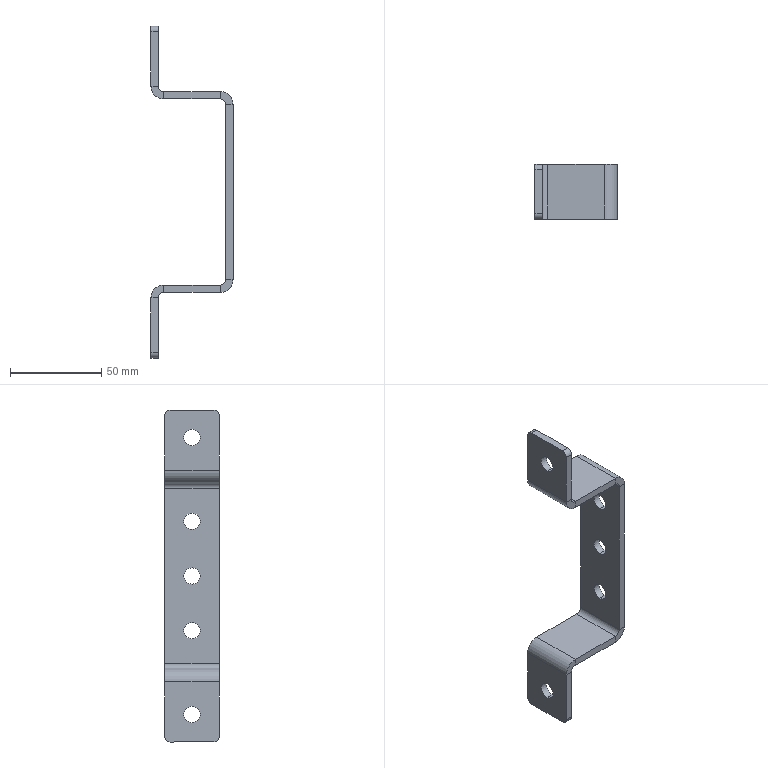Component | SolidWorks | OutputN01400AType40001100-3 | 1 solid | 52 faces | volume 29347 mm3 | plane 30 | cylinder 22 | commonest cylinder face diameters 9 x10 6 x8 14 x4